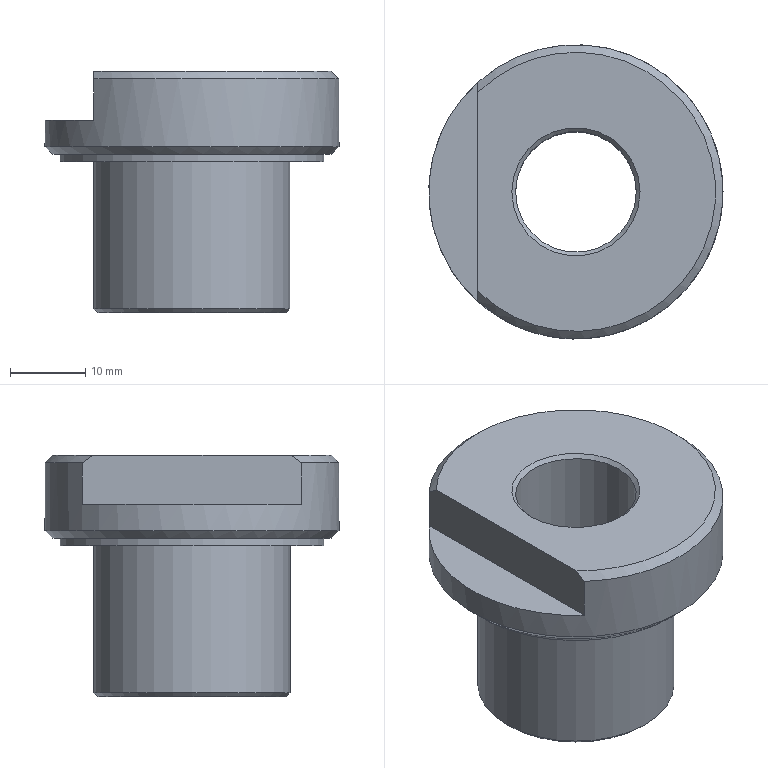Component | NX | DRILL_BUSHING | 1 solid | 17 faces | box 39 x 39 x 32 mm | volume 17133 mm3 | plane 7 | cylinder 5 | cone 5 | commonest cylinder face diameters 35 x1 39 x1 30 x1 26 x1 16 x1
STEP:
#1=CARTESIAN_POINT('',(0.,0.,0.));
#2=DIRECTION('',(0.,0.,1.));
#3=DIRECTION('',(1.,0.,0.));
#4=AXIS2_PLACEMENT_3D('',#1,#2,#3);
#5=CARTESIAN_POINT('',(30.5,0.,39.));
#6=VERTEX_POINT('',#5);
#7=CARTESIAN_POINT('',(13.,0.,39.));
#8=DIRECTION('',(0.,0.,1.));
#9=DIRECTION('',(1.,0.,0.));
#10=AXIS2_PLACEMENT_3D('',#7,#8,#9);
#11=CIRCLE('',#10,17.5);
#12=CARTESIAN_POINT('',(13.,0.,39.));
#13=DIRECTION('',(0.,0.,-1.));
#14=DIRECTION('',(-1.,0.,0.));
#15=AXIS2_PLACEMENT_3D('',#12,#13,#14);
#16=CYLINDRICAL_SURFACE('',#15,17.5);
#17=CARTESIAN_POINT('',(9.425,0.));
#18=DIRECTION('',(-1.,0.));
#19=VECTOR('',#18,1.);
#20=LINE('',#17,#19);
#21=(GEOMETRIC_REPRESENTATION_CONTEXT(2)PARAMETRIC_REPRESENTATION_CONTEXT()REPRESENTATION_CONTEXT('',''));
#22=DEFINITIONAL_REPRESENTATION('',(#20),#21);
#23=PCURVE('',#16,#22);
#24=CARTESIAN_POINT('',(13.,0.,39.));
#25=DIRECTION('',(0.,0.,1.));
#26=DIRECTION('',(1.,0.,0.));
#27=AXIS2_PLACEMENT_3D('',#24,#25,#26);
#28=PLANE('',#27);
#29=CARTESIAN_POINT('',(0.,0.));
#30=DIRECTION('',(1.,0.));
#31=AXIS2_PLACEMENT_2D('',#29,#30);
#32=CIRCLE('',#31,17.5);
#33=(GEOMETRIC_REPRESENTATION_CONTEXT(2)PARAMETRIC_REPRESENTATION_CONTEXT()REPRESENTATION_CONTEXT('',''));
#34=DEFINITIONAL_REPRESENTATION('',(#32),#33);
#35=PCURVE('',#28,#34);
#36=SURFACE_CURVE('',#11,(#23,#35),.PCURVE_S1.);
#37=EDGE_CURVE('',#6,#6,#36,.T.);
#38=ORIENTED_EDGE('',*,*,#37,.F.);
#39=CARTESIAN_POINT('',(30.5,0.,38.));
#40=VERTEX_POINT('',#39);
#41=CARTESIAN_POINT('',(30.5,0.,39.));
#42=CARTESIAN_POINT('',(30.5,0.,38.));
#43=B_SPLINE_CURVE_WITH_KNOTS('',1,(#41,#42),.UNSPECIFIED.,.F.,.F.,(2,2),(0.,1.),.PIECEWISE_BEZIER_KNOTS.);
#44=CARTESIAN_POINT('',(9.425,0.));
#45=DIRECTION('',(0.,1.));
#46=VECTOR('',#45,1.);
#47=LINE('',#44,#46);
#48=(GEOMETRIC_REPRESENTATION_CONTEXT(2)PARAMETRIC_REPRESENTATION_CONTEXT()REPRESENTATION_CONTEXT('',''));
#49=DEFINITIONAL_REPRESENTATION('',(#47),#48);
#50=PCURVE('',#16,#49);
#51=CARTESIAN_POINT('',(3.142,0.));
#52=DIRECTION('',(0.,1.));
#53=VECTOR('',#52,1.);
#54=LINE('',#51,#53);
#55=(GEOMETRIC_REPRESENTATION_CONTEXT(2)PARAMETRIC_REPRESENTATION_CONTEXT()REPRESENTATION_CONTEXT('',''));
#56=DEFINITIONAL_REPRESENTATION('',(#54),#55);
#57=PCURVE('',#16,#56);
#58=SEAM_CURVE('',#43,(#50,#57),.PCURVE_S1.);
#59=EDGE_CURVE('',#6,#40,#58,.T.);
#60=ORIENTED_EDGE('',*,*,#59,.T.);
#61=CARTESIAN_POINT('',(13.,0.,38.));
#62=DIRECTION('',(0.,0.,1.));
#63=DIRECTION('',(1.,0.,0.));
#64=AXIS2_PLACEMENT_3D('',#61,#62,#63);
#65=CIRCLE('',#64,17.5);
#66=CARTESIAN_POINT('',(9.425,1.));
#67=DIRECTION('',(-1.,0.));
#68=VECTOR('',#67,1.);
#69=LINE('',#66,#68);
#70=(GEOMETRIC_REPRESENTATION_CONTEXT(2)PARAMETRIC_REPRESENTATION_CONTEXT()REPRESENTATION_CONTEXT('',''));
#71=DEFINITIONAL_REPRESENTATION('',(#69),#70);
#72=PCURVE('',#16,#71);
#73=CARTESIAN_POINT('',(13.,0.,38.));
#74=DIRECTION('',(0.,0.,1.));
#75=DIRECTION('',(1.,0.,0.));
#76=AXIS2_PLACEMENT_3D('',#73,#74,#75);
#77=PLANE('',#76);
#78=CARTESIAN_POINT('',(0.,0.));
#79=DIRECTION('',(1.,0.));
#80=AXIS2_PLACEMENT_2D('',#78,#79);
#81=CIRCLE('',#80,17.5);
#82=(GEOMETRIC_REPRESENTATION_CONTEXT(2)PARAMETRIC_REPRESENTATION_CONTEXT()REPRESENTATION_CONTEXT('',''));
#83=DEFINITIONAL_REPRESENTATION('',(#81),#82);
#84=PCURVE('',#77,#83);
#85=SURFACE_CURVE('',#65,(#72,#84),.PCURVE_S1.);
#86=EDGE_CURVE('',#40,#40,#85,.T.);
#87=ORIENTED_EDGE('',*,*,#86,.T.);
#88=ORIENTED_EDGE('',*,*,#59,.F.);
#89=EDGE_LOOP('',(#38,#60,#87,#88));
#90=FACE_BOUND('',#89,.T.);
#91=ADVANCED_FACE('',(#90),#16,.T.);
#92=CARTESIAN_POINT('',(28.,0.,38.));
#93=VERTEX_POINT('',#92);
#94=CARTESIAN_POINT('',(13.,0.,38.));
#95=DIRECTION('',(0.,0.,-1.));
#96=DIRECTION('',(1.,0.,0.));
#97=AXIS2_PLACEMENT_3D('',#94,#95,#96);
#98=CIRCLE('',#97,15.);
#99=CARTESIAN_POINT('',(15.,0.));
#100=CARTESIAN_POINT('',(15.,-25.981));
#101=CARTESIAN_POINT('',(-7.5,-12.99));
#102=CARTESIAN_POINT('',(-30.,-0.));
#103=CARTESIAN_POINT('',(-7.5,12.99));
#104=CARTESIAN_POINT('',(15.,25.981));
#105=CARTESIAN_POINT('',(15.,0.));
#106=(BOUNDED_CURVE()B_SPLINE_CURVE(2,(#99,#100,#101,#102,#103,#104,#105),.UNSPECIFIED.,.T.,.F.)B_SPLINE_CURVE_WITH_KNOTS((1,2,2,2,2,1),(-2.094,0.,2.094,4.189,6.283,8.378),.UNSPECIFIED.)CURVE()GEOMETRIC_REPRESENTATION_ITEM()RATIONAL_B_SPLINE_CURVE((1.,0.5,1.,0.5,1.,0.5,1.))REPRESENTATION_ITEM(''));
#107=(GEOMETRIC_REPRESENTATION_CONTEXT(2)PARAMETRIC_REPRESENTATION_CONTEXT()REPRESENTATION_CONTEXT('',''));
#108=DEFINITIONAL_REPRESENTATION('',(#106),#107);
#109=PCURVE('',#77,#108);
#110=CARTESIAN_POINT('',(13.,0.,38.));
#111=DIRECTION('',(0.,0.,1.));
#112=DIRECTION('',(1.,0.,0.));
#113=AXIS2_PLACEMENT_3D('',#110,#111,#112);
#114=CYLINDRICAL_SURFACE('',#113,15.);
#115=CARTESIAN_POINT('',(6.283,0.));
#116=DIRECTION('',(-1.,0.));
#117=VECTOR('',#116,1.);
#118=LINE('',#115,#117);
#119=(GEOMETRIC_REPRESENTATION_CONTEXT(2)PARAMETRIC_REPRESENTATION_CONTEXT()REPRESENTATION_CONTEXT('',''));
#120=DEFINITIONAL_REPRESENTATION('',(#118),#119);
#121=PCURVE('',#114,#120);
#122=SURFACE_CURVE('',#98,(#109,#121),.PCURVE_S1.);
#123=EDGE_CURVE('',#93,#93,#122,.T.);
#124=ORIENTED_EDGE('',*,*,#123,.F.);
#125=EDGE_LOOP('',(#124));
#126=FACE_BOUND('',#125,.T.);
#127=ORIENTED_EDGE('',*,*,#86,.F.);
#128=EDGE_LOOP('',(#127));
#129=FACE_BOUND('',#128,.T.);
#130=ADVANCED_FACE('',(#126,#129),#77,.F.);
#131=CARTESIAN_POINT('',(32.5,0.,40.));
#132=VERTEX_POINT('',#131);
#133=CARTESIAN_POINT('',(-0.,14.534,40.));
#134=VERTEX_POINT('',#133);
#135=CARTESIAN_POINT('',(13.,0.,40.));
#136=DIRECTION('',(0.,0.,1.));
#137=DIRECTION('',(1.,0.,0.));
#138=AXIS2_PLACEMENT_3D('',#135,#136,#137);
#139=CIRCLE('',#138,19.5);
#140=CARTESIAN_POINT('',(13.,0.,50.));
#141=DIRECTION('',(0.,0.,-1.));
#142=DIRECTION('',(-1.,0.,0.));
#143=AXIS2_PLACEMENT_3D('',#140,#141,#142);
#144=CYLINDRICAL_SURFACE('',#143,19.5);
#145=CARTESIAN_POINT('',(3.142,10.));
#146=DIRECTION('',(-1.,0.));
#147=VECTOR('',#146,1.);
#148=LINE('',#145,#147);
#149=(GEOMETRIC_REPRESENTATION_CONTEXT(2)PARAMETRIC_REPRESENTATION_CONTEXT()REPRESENTATION_CONTEXT('',''));
#150=DEFINITIONAL_REPRESENTATION('',(#148),#149);
#151=PCURVE('',#144,#150);
#152=CARTESIAN_POINT('',(13.,0.,40.));
#153=DIRECTION('',(0.,0.,1.));
#154=DIRECTION('',(1.,0.,0.));
#155=AXIS2_PLACEMENT_3D('',#152,#153,#154);
#156=CONICAL_SURFACE('',#155,19.5,0.7854);
#157=CARTESIAN_POINT('',(0.,0.));
#158=DIRECTION('',(1.,0.));
#159=VECTOR('',#158,1.);
#160=LINE('',#157,#159);
#161=(GEOMETRIC_REPRESENTATION_CONTEXT(2)PARAMETRIC_REPRESENTATION_CONTEXT()REPRESENTATION_CONTEXT('',''));
#162=DEFINITIONAL_REPRESENTATION('',(#160),#161);
#163=PCURVE('',#156,#162);
#164=SURFACE_CURVE('',#139,(#151,#163),.PCURVE_S1.);
#165=EDGE_CURVE('',#132,#134,#164,.T.);
#166=ORIENTED_EDGE('',*,*,#165,.T.);
#167=CARTESIAN_POINT('',(0.,14.534,43.5));
#168=VERTEX_POINT('',#167);
#169=CARTESIAN_POINT('',(-0.,14.534,43.5));
#170=CARTESIAN_POINT('',(-0.,14.534,40.));
#171=B_SPLINE_CURVE_WITH_KNOTS('',1,(#169,#170),.UNSPECIFIED.,.F.,.F.,(2,2),(6.5,10.),.PIECEWISE_BEZIER_KNOTS.);
#172=CARTESIAN_POINT('',(0.8411,0.));
#173=DIRECTION('',(0.,1.));
#174=VECTOR('',#173,1.);
#175=LINE('',#172,#174);
#176=(GEOMETRIC_REPRESENTATION_CONTEXT(2)PARAMETRIC_REPRESENTATION_CONTEXT()REPRESENTATION_CONTEXT('',''));
#177=DEFINITIONAL_REPRESENTATION('',(#175),#176);
#178=PCURVE('',#144,#177);
#179=CARTESIAN_POINT('',(7.124,0.));
#180=DIRECTION('',(0.,1.));
#181=VECTOR('',#180,1.);
#182=LINE('',#179,#181);
#183=(GEOMETRIC_REPRESENTATION_CONTEXT(2)PARAMETRIC_REPRESENTATION_CONTEXT()REPRESENTATION_CONTEXT('',''));
#184=DEFINITIONAL_REPRESENTATION('',(#182),#183);
#185=PCURVE('',#144,#184);
#186=SEAM_CURVE('',#171,(#178,#185),.PCURVE_S1.);
#187=EDGE_CURVE('',#168,#134,#186,.T.);
#188=ORIENTED_EDGE('',*,*,#187,.F.);
#189=CARTESIAN_POINT('',(0.,14.534,49.));
#190=VERTEX_POINT('',#189);
#191=CARTESIAN_POINT('',(0.,14.534,50.));
#192=DIRECTION('',(0.,0.,1.));
#193=VECTOR('',#192,1.);
#194=LINE('',#191,#193);
#195=CARTESIAN_POINT('',(0.8411,0.));
#196=DIRECTION('',(0.,-1.));
#197=VECTOR('',#196,1.);
#198=LINE('',#195,#197);
#199=(GEOMETRIC_REPRESENTATION_CONTEXT(2)PARAMETRIC_REPRESENTATION_CONTEXT()REPRESENTATION_CONTEXT('',''));
#200=DEFINITIONAL_REPRESENTATION('',(#198),#199);
#201=PCURVE('',#144,#200);
#202=CARTESIAN_POINT('',(0.,-23.,43.5));
#203=DIRECTION('',(1.,0.,0.));
#204=DIRECTION('',(-0.,1.,0.));
#205=AXIS2_PLACEMENT_3D('',#202,#203,#204);
#206=PLANE('',#205);
#207=CARTESIAN_POINT('',(37.534,6.5));
#208=DIRECTION('',(0.,1.));
#209=VECTOR('',#208,1.);
#210=LINE('',#207,#209);
#211=(GEOMETRIC_REPRESENTATION_CONTEXT(2)PARAMETRIC_REPRESENTATION_CONTEXT()REPRESENTATION_CONTEXT('',''));
#212=DEFINITIONAL_REPRESENTATION('',(#210),#211);
#213=PCURVE('',#206,#212);
#214=SURFACE_CURVE('',#194,(#201,#213),.PCURVE_S1.);
#215=EDGE_CURVE('',#168,#190,#214,.T.);
#216=ORIENTED_EDGE('',*,*,#215,.T.);
#217=CARTESIAN_POINT('',(0.,-14.534,49.));
#218=VERTEX_POINT('',#217);
#219=CARTESIAN_POINT('',(13.,0.,49.));
#220=DIRECTION('',(0.,0.,-1.));
#221=DIRECTION('',(1.,0.,0.));
#222=AXIS2_PLACEMENT_3D('',#219,#220,#221);
#223=CIRCLE('',#222,19.5);
#224=CARTESIAN_POINT('',(-3.142,1.));
#225=DIRECTION('',(1.,0.));
#226=VECTOR('',#225,1.);
#227=LINE('',#224,#226);
#228=(GEOMETRIC_REPRESENTATION_CONTEXT(2)PARAMETRIC_REPRESENTATION_CONTEXT()REPRESENTATION_CONTEXT('',''));
#229=DEFINITIONAL_REPRESENTATION('',(#227),#228);
#230=PCURVE('',#144,#229);
#231=CARTESIAN_POINT('',(13.,0.,50.));
#232=DIRECTION('',(0.,0.,-1.));
#233=DIRECTION('',(-1.,0.,0.));
#234=AXIS2_PLACEMENT_3D('',#231,#232,#233);
#235=CONICAL_SURFACE('',#234,18.5,0.7854);
#236=CARTESIAN_POINT('',(-3.142,1.));
#237=DIRECTION('',(1.,0.));
#238=VECTOR('',#237,1.);
#239=LINE('',#236,#238);
#240=(GEOMETRIC_REPRESENTATION_CONTEXT(2)PARAMETRIC_REPRESENTATION_CONTEXT()REPRESENTATION_CONTEXT('',''));
#241=DEFINITIONAL_REPRESENTATION('',(#239),#240);
#242=PCURVE('',#235,#241);
#243=SURFACE_CURVE('',#223,(#230,#242),.PCURVE_S1.);
#244=EDGE_CURVE('',#190,#218,#243,.T.);
#245=ORIENTED_EDGE('',*,*,#244,.T.);
#246=CARTESIAN_POINT('',(0.,-14.534,43.5));
#247=VERTEX_POINT('',#246);
#248=CARTESIAN_POINT('',(0.,-14.534,50.));
#249=DIRECTION('',(0.,0.,-1.));
#250=VECTOR('',#249,1.);
#251=LINE('',#248,#250);
#252=CARTESIAN_POINT('',(5.442,0.));
#253=DIRECTION('',(0.,1.));
#254=VECTOR('',#253,1.);
#255=LINE('',#252,#254);
#256=(GEOMETRIC_REPRESENTATION_CONTEXT(2)PARAMETRIC_REPRESENTATION_CONTEXT()REPRESENTATION_CONTEXT('',''));
#257=DEFINITIONAL_REPRESENTATION('',(#255),#256);
#258=PCURVE('',#144,#257);
#259=CARTESIAN_POINT('',(8.466,6.5));
#260=DIRECTION('',(0.,-1.));
#261=VECTOR('',#260,1.);
#262=LINE('',#259,#261);
#263=(GEOMETRIC_REPRESENTATION_CONTEXT(2)PARAMETRIC_REPRESENTATION_CONTEXT()REPRESENTATION_CONTEXT('',''));
#264=DEFINITIONAL_REPRESENTATION('',(#262),#263);
#265=PCURVE('',#206,#264);
#266=SURFACE_CURVE('',#251,(#258,#265),.PCURVE_S1.);
#267=EDGE_CURVE('',#218,#247,#266,.T.);
#268=ORIENTED_EDGE('',*,*,#267,.T.);
#269=CARTESIAN_POINT('',(13.,0.,43.5));
#270=DIRECTION('',(0.,0.,1.));
#271=DIRECTION('',(1.,0.,0.));
#272=AXIS2_PLACEMENT_3D('',#269,#270,#271);
#273=CIRCLE('',#272,19.5);
#274=CARTESIAN_POINT('',(9.425,6.5));
#275=DIRECTION('',(-1.,0.));
#276=VECTOR('',#275,1.);
#277=LINE('',#274,#276);
#278=(GEOMETRIC_REPRESENTATION_CONTEXT(2)PARAMETRIC_REPRESENTATION_CONTEXT()REPRESENTATION_CONTEXT('',''));
#279=DEFINITIONAL_REPRESENTATION('',(#277),#278);
#280=PCURVE('',#144,#279);
#281=CARTESIAN_POINT('',(13.,0.,43.5));
#282=DIRECTION('',(0.,0.,1.));
#283=DIRECTION('',(1.,0.,0.));
#284=AXIS2_PLACEMENT_3D('',#281,#282,#283);
#285=PLANE('',#284);
#286=CARTESIAN_POINT('',(0.,0.));
#287=DIRECTION('',(1.,0.));
#288=AXIS2_PLACEMENT_2D('',#286,#287);
#289=CIRCLE('',#288,19.5);
#290=(GEOMETRIC_REPRESENTATION_CONTEXT(2)PARAMETRIC_REPRESENTATION_CONTEXT()REPRESENTATION_CONTEXT('',''));
#291=DEFINITIONAL_REPRESENTATION('',(#289),#290);
#292=PCURVE('',#285,#291);
#293=SURFACE_CURVE('',#273,(#280,#292),.PCURVE_S1.);
#294=EDGE_CURVE('',#168,#247,#293,.T.);
#295=ORIENTED_EDGE('',*,*,#294,.F.);
#296=ORIENTED_EDGE('',*,*,#187,.T.);
#297=CARTESIAN_POINT('',(13.,0.,40.));
#298=DIRECTION('',(0.,0.,1.));
#299=DIRECTION('',(1.,0.,0.));
#300=AXIS2_PLACEMENT_3D('',#297,#298,#299);
#301=CIRCLE('',#300,19.5);
#302=CARTESIAN_POINT('',(9.425,10.));
#303=DIRECTION('',(-1.,0.));
#304=VECTOR('',#303,1.);
#305=LINE('',#302,#304);
#306=(GEOMETRIC_REPRESENTATION_CONTEXT(2)PARAMETRIC_REPRESENTATION_CONTEXT()REPRESENTATION_CONTEXT('',''));
#307=DEFINITIONAL_REPRESENTATION('',(#305),#306);
#308=PCURVE('',#144,#307);
#309=CARTESIAN_POINT('',(0.,0.));
#310=DIRECTION('',(1.,0.));
#311=VECTOR('',#310,1.);
#312=LINE('',#309,#311);
#313=(GEOMETRIC_REPRESENTATION_CONTEXT(2)PARAMETRIC_REPRESENTATION_CONTEXT()REPRESENTATION_CONTEXT('',''));
#314=DEFINITIONAL_REPRESENTATION('',(#312),#313);
#315=PCURVE('',#156,#314);
#316=SURFACE_CURVE('',#301,(#308,#315),.PCURVE_S1.);
#317=EDGE_CURVE('',#134,#132,#316,.T.);
#318=ORIENTED_EDGE('',*,*,#317,.T.);
#319=EDGE_LOOP('',(#166,#188,#216,#245,#268,#295,#296,#318));
#320=FACE_BOUND('',#319,.T.);
#321=ADVANCED_FACE('',(#320),#144,.T.);
#322=CARTESIAN_POINT('',(21.5,0.,50.));
#323=VERTEX_POINT('',#322);
#324=CARTESIAN_POINT('',(13.,0.,50.));
#325=DIRECTION('',(0.,0.,-1.));
#326=DIRECTION('',(1.,0.,0.));
#327=AXIS2_PLACEMENT_3D('',#324,#325,#326);
#328=CIRCLE('',#327,8.5);
#329=CARTESIAN_POINT('',(13.,0.,50.));
#330=DIRECTION('',(0.,0.,1.));
#331=DIRECTION('',(1.,0.,0.));
#332=AXIS2_PLACEMENT_3D('',#329,#330,#331);
#333=PLANE('',#332);
#334=CARTESIAN_POINT('',(8.5,0.));
#335=CARTESIAN_POINT('',(8.5,-14.722));
#336=CARTESIAN_POINT('',(-4.25,-7.361));
#337=CARTESIAN_POINT('',(-17.,-0.));
#338=CARTESIAN_POINT('',(-4.25,7.361));
#339=CARTESIAN_POINT('',(8.5,14.722));
#340=CARTESIAN_POINT('',(8.5,0.));
#341=(BOUNDED_CURVE()B_SPLINE_CURVE(2,(#334,#335,#336,#337,#338,#339,#340),.UNSPECIFIED.,.T.,.F.)B_SPLINE_CURVE_WITH_KNOTS((1,2,2,2,2,1),(-2.094,0.,2.094,4.189,6.283,8.378),.UNSPECIFIED.)CURVE()GEOMETRIC_REPRESENTATION_ITEM()RATIONAL_B_SPLINE_CURVE((1.,0.5,1.,0.5,1.,0.5,1.))REPRESENTATION_ITEM(''));
#342=(GEOMETRIC_REPRESENTATION_CONTEXT(2)PARAMETRIC_REPRESENTATION_CONTEXT()REPRESENTATION_CONTEXT('',''));
#343=DEFINITIONAL_REPRESENTATION('',(#341),#342);
#344=PCURVE('',#333,#343);
#345=CARTESIAN_POINT('',(13.,0.,50.));
#346=DIRECTION('',(0.,0.,1.));
#347=DIRECTION('',(1.,0.,0.));
#348=AXIS2_PLACEMENT_3D('',#345,#346,#347);
#349=CONICAL_SURFACE('',#348,8.5,0.7854);
#350=CARTESIAN_POINT('',(6.283,0.));
#351=DIRECTION('',(-1.,0.));
#352=VECTOR('',#351,1.);
#353=LINE('',#350,#352);
#354=(GEOMETRIC_REPRESENTATION_CONTEXT(2)PARAMETRIC_REPRESENTATION_CONTEXT()REPRESENTATION_CONTEXT('',''));
#355=DEFINITIONAL_REPRESENTATION('',(#353),#354);
#356=PCURVE('',#349,#355);
#357=SURFACE_CURVE('',#328,(#344,#356),.PCURVE_S1.);
#358=EDGE_CURVE('',#323,#323,#357,.T.);
#359=ORIENTED_EDGE('',*,*,#358,.T.);
#360=EDGE_LOOP('',(#359));
#361=FACE_BOUND('',#360,.T.);
#362=CARTESIAN_POINT('',(0.,-13.162,50.));
#363=VERTEX_POINT('',#362);
#364=CARTESIAN_POINT('',(0.,13.162,50.));
#365=VERTEX_POINT('',#364);
#366=CARTESIAN_POINT('',(0.,-23.,50.));
#367=DIRECTION('',(-0.,1.,0.));
#368=VECTOR('',#367,1.);
#369=LINE('',#366,#368);
#370=CARTESIAN_POINT('',(-13.,-23.));
#371=DIRECTION('',(-0.,1.));
#372=VECTOR('',#371,1.);
#373=LINE('',#370,#372);
#374=(GEOMETRIC_REPRESENTATION_CONTEXT(2)PARAMETRIC_REPRESENTATION_CONTEXT()REPRESENTATION_CONTEXT('',''));
#375=DEFINITIONAL_REPRESENTATION('',(#373),#374);
#376=PCURVE('',#333,#375);
#377=CARTESIAN_POINT('',(0.,6.5));
#378=DIRECTION('',(1.,0.));
#379=VECTOR('',#378,1.);
#380=LINE('',#377,#379);
#381=(GEOMETRIC_REPRESENTATION_CONTEXT(2)PARAMETRIC_REPRESENTATION_CONTEXT()REPRESENTATION_CONTEXT('',''));
#382=DEFINITIONAL_REPRESENTATION('',(#380),#381);
#383=PCURVE('',#206,#382);
#384=SURFACE_CURVE('',#369,(#376,#383),.PCURVE_S1.);
#385=EDGE_CURVE('',#363,#365,#384,.T.);
#386=ORIENTED_EDGE('',*,*,#385,.F.);
#387=CARTESIAN_POINT('',(13.,0.,50.));
#388=DIRECTION('',(0.,0.,1.));
#389=DIRECTION('',(1.,0.,0.));
#390=AXIS2_PLACEMENT_3D('',#387,#388,#389);
#391=CIRCLE('',#390,18.5);
#392=CARTESIAN_POINT('',(0.,0.));
#393=DIRECTION('',(1.,0.));
#394=AXIS2_PLACEMENT_2D('',#392,#393);
#395=CIRCLE('',#394,18.5);
#396=(GEOMETRIC_REPRESENTATION_CONTEXT(2)PARAMETRIC_REPRESENTATION_CONTEXT()REPRESENTATION_CONTEXT('',''));
#397=DEFINITIONAL_REPRESENTATION('',(#395),#396);
#398=PCURVE('',#333,#397);
#399=CARTESIAN_POINT('',(9.425,0.));
#400=DIRECTION('',(-1.,0.));
#401=VECTOR('',#400,1.);
#402=LINE('',#399,#401);
#403=(GEOMETRIC_REPRESENTATION_CONTEXT(2)PARAMETRIC_REPRESENTATION_CONTEXT()REPRESENTATION_CONTEXT('',''));
#404=DEFINITIONAL_REPRESENTATION('',(#402),#403);
#405=PCURVE('',#235,#404);
#406=SURFACE_CURVE('',#391,(#398,#405),.PCURVE_S1.);
#407=EDGE_CURVE('',#363,#365,#406,.T.);
#408=ORIENTED_EDGE('',*,*,#407,.T.);
#409=EDGE_LOOP('',(#386,#408));
#410=FACE_BOUND('',#409,.T.);
#411=ADVANCED_FACE('',(#361,#410),#333,.T.);
#412=CARTESIAN_POINT('',(31.5,0.,39.));
#413=VERTEX_POINT('',#412);
#414=CARTESIAN_POINT('',(13.,0.,39.));
#415=DIRECTION('',(0.,0.,-1.));
#416=DIRECTION('',(1.,0.,0.));
#417=AXIS2_PLACEMENT_3D('',#414,#415,#416);
#418=CIRCLE('',#417,18.5);
#419=CARTESIAN_POINT('',(18.5,0.));
#420=CARTESIAN_POINT('',(18.5,-32.043));
#421=CARTESIAN_POINT('',(-9.25,-16.021));
#422=CARTESIAN_POINT('',(-37.,-0.));
#423=CARTESIAN_POINT('',(-9.25,16.021));
#424=CARTESIAN_POINT('',(18.5,32.043));
#425=CARTESIAN_POINT('',(18.5,0.));
#426=(BOUNDED_CURVE()B_SPLINE_CURVE(2,(#419,#420,#421,#422,#423,#424,#425),.UNSPECIFIED.,.T.,.F.)B_SPLINE_CURVE_WITH_KNOTS((1,2,2,2,2,1),(-2.094,0.,2.094,4.189,6.283,8.378),.UNSPECIFIED.)CURVE()GEOMETRIC_REPRESENTATION_ITEM()RATIONAL_B_SPLINE_CURVE((1.,0.5,1.,0.5,1.,0.5,1.))REPRESENTATION_ITEM(''));
#427=(GEOMETRIC_REPRESENTATION_CONTEXT(2)PARAMETRIC_REPRESENTATION_CONTEXT()REPRESENTATION_CONTEXT('',''));
#428=DEFINITIONAL_REPRESENTATION('',(#426),#427);
#429=PCURVE('',#28,#428);
#430=CARTESIAN_POINT('',(6.283,-1.));
#431=DIRECTION('',(-1.,0.));
#432=VECTOR('',#431,1.);
#433=LINE('',#430,#432);
#434=(GEOMETRIC_REPRESENTATION_CONTEXT(2)PARAMETRIC_REPRESENTATION_CONTEXT()REPRESENTATION_CONTEXT('',''));
#435=DEFINITIONAL_REPRESENTATION('',(#433),#434);
#436=PCURVE('',#156,#435);
#437=SURFACE_CURVE('',#418,(#429,#436),.PCURVE_S1.);
#438=EDGE_CURVE('',#413,#413,#437,.T.);
#439=ORIENTED_EDGE('',*,*,#438,.T.);
#440=EDGE_LOOP('',(#439));
#441=FACE_BOUND('',#440,.T.);
#442=ORIENTED_EDGE('',*,*,#37,.T.);
#443=EDGE_LOOP('',(#442));
#444=FACE_BOUND('',#443,.T.);
#445=ADVANCED_FACE('',(#441,#444),#28,.F.);
#446=CARTESIAN_POINT('',(28.,0.,39.));
#447=VERTEX_POINT('',#446);
#448=CARTESIAN_POINT('',(13.,0.,39.));
#449=DIRECTION('',(0.,0.,1.));
#450=DIRECTION('',(1.,0.,0.));
#451=AXIS2_PLACEMENT_3D('',#448,#449,#450);
#452=CIRCLE('',#451,15.);
#453=CARTESIAN_POINT('',(13.,0.,39.));
#454=DIRECTION('',(0.,0.,1.));
#455=DIRECTION('',(1.,0.,0.));
#456=AXIS2_PLACEMENT_3D('',#453,#454,#455);
#457=PLANE('',#456);
#458=CARTESIAN_POINT('',(0.,0.));
#459=DIRECTION('',(1.,0.));
#460=AXIS2_PLACEMENT_2D('',#458,#459);
#461=CIRCLE('',#460,15.);
#462=(GEOMETRIC_REPRESENTATION_CONTEXT(2)PARAMETRIC_REPRESENTATION_CONTEXT()REPRESENTATION_CONTEXT('',''));
#463=DEFINITIONAL_REPRESENTATION('',(#461),#462);
#464=PCURVE('',#457,#463);
#465=CARTESIAN_POINT('',(0.,1.));
#466=DIRECTION('',(1.,0.));
#467=VECTOR('',#466,1.);
#468=LINE('',#465,#467);
#469=(GEOMETRIC_REPRESENTATION_CONTEXT(2)PARAMETRIC_REPRESENTATION_CONTEXT()REPRESENTATION_CONTEXT('',''));
#470=DEFINITIONAL_REPRESENTATION('',(#468),#469);
#471=PCURVE('',#114,#470);
#472=SURFACE_CURVE('',#452,(#464,#471),.PCURVE_S1.);
#473=EDGE_CURVE('',#447,#447,#472,.T.);
#474=ORIENTED_EDGE('',*,*,#473,.F.);
#475=EDGE_LOOP('',(#474));
#476=FACE_BOUND('',#475,.T.);
#477=CARTESIAN_POINT('',(26.,0.,39.));
#478=VERTEX_POINT('',#477);
#479=CARTESIAN_POINT('',(13.,0.,39.));
#480=DIRECTION('',(0.,0.,-1.));
#481=DIRECTION('',(1.,0.,0.));
#482=AXIS2_PLACEMENT_3D('',#479,#480,#481);
#483=CIRCLE('',#482,13.);
#484=CARTESIAN_POINT('',(13.,0.));
#485=CARTESIAN_POINT('',(13.,-22.517));
#486=CARTESIAN_POINT('',(-6.5,-11.258));
#487=CARTESIAN_POINT('',(-26.,-0.));
#488=CARTESIAN_POINT('',(-6.5,11.258));
#489=CARTESIAN_POINT('',(13.,22.517));
#490=CARTESIAN_POINT('',(13.,0.));
#491=(BOUNDED_CURVE()B_SPLINE_CURVE(2,(#484,#485,#486,#487,#488,#489,#490),.UNSPECIFIED.,.T.,.F.)B_SPLINE_CURVE_WITH_KNOTS((1,2,2,2,2,1),(-2.094,0.,2.094,4.189,6.283,8.378),.UNSPECIFIED.)CURVE()GEOMETRIC_REPRESENTATION_ITEM()RATIONAL_B_SPLINE_CURVE((1.,0.5,1.,0.5,1.,0.5,1.))REPRESENTATION_ITEM(''));
#492=(GEOMETRIC_REPRESENTATION_CONTEXT(2)PARAMETRIC_REPRESENTATION_CONTEXT()REPRESENTATION_CONTEXT('',''));
#493=DEFINITIONAL_REPRESENTATION('',(#491),#492);
#494=PCURVE('',#457,#493);
#495=CARTESIAN_POINT('',(13.,0.,38.));
#496=DIRECTION('',(0.,0.,-1.));
#497=DIRECTION('',(-1.,0.,0.));
#498=AXIS2_PLACEMENT_3D('',#495,#496,#497);
#499=CYLINDRICAL_SURFACE('',#498,13.);
#500=CARTESIAN_POINT('',(3.142,-1.));
#501=DIRECTION('',(1.,0.));
#502=VECTOR('',#501,1.);
#503=LINE('',#500,#502);
#504=(GEOMETRIC_REPRESENTATION_CONTEXT(2)PARAMETRIC_REPRESENTATION_CONTEXT()REPRESENTATION_CONTEXT('',''));
#505=DEFINITIONAL_REPRESENTATION('',(#503),#504);
#506=PCURVE('',#499,#505);
#507=SURFACE_CURVE('',#483,(#494,#506),.PCURVE_S1.);
#508=EDGE_CURVE('',#478,#478,#507,.T.);
#509=ORIENTED_EDGE('',*,*,#508,.F.);
#510=EDGE_LOOP('',(#509));
#511=FACE_BOUND('',#510,.T.);
#512=ADVANCED_FACE('',(#476,#511),#457,.F.);
#513=ORIENTED_EDGE('',*,*,#123,.F.);
#514=CARTESIAN_POINT('',(28.,0.,38.));
#515=CARTESIAN_POINT('',(28.,0.,39.));
#516=B_SPLINE_CURVE_WITH_KNOTS('',1,(#514,#515),.UNSPECIFIED.,.F.,.F.,(2,2),(0.,1.),.PIECEWISE_BEZIER_KNOTS.);
#517=CARTESIAN_POINT('',(6.283,0.));
#518=DIRECTION('',(0.,1.));
#519=VECTOR('',#518,1.);
#520=LINE('',#517,#519);
#521=(GEOMETRIC_REPRESENTATION_CONTEXT(2)PARAMETRIC_REPRESENTATION_CONTEXT()REPRESENTATION_CONTEXT('',''));
#522=DEFINITIONAL_REPRESENTATION('',(#520),#521);
#523=PCURVE('',#114,#522);
#524=CARTESIAN_POINT('',(0.,0.));
#525=DIRECTION('',(0.,1.));
#526=VECTOR('',#525,1.);
#527=LINE('',#524,#526);
#528=(GEOMETRIC_REPRESENTATION_CONTEXT(2)PARAMETRIC_REPRESENTATION_CONTEXT()REPRESENTATION_CONTEXT('',''));
#529=DEFINITIONAL_REPRESENTATION('',(#527),#528);
#530=PCURVE('',#114,#529);
#531=SEAM_CURVE('',#516,(#523,#530),.PCURVE_S1.);
#532=EDGE_CURVE('',#93,#447,#531,.T.);
#533=ORIENTED_EDGE('',*,*,#532,.T.);
#534=ORIENTED_EDGE('',*,*,#473,.F.);
#535=ORIENTED_EDGE('',*,*,#532,.F.);
#536=EDGE_LOOP('',(#513,#533,#534,#535));
#537=FACE_BOUND('',#536,.F.);
#538=ADVANCED_FACE('',(#537),#114,.F.);
#539=CARTESIAN_POINT('',(21.5,0.,18.));
#540=VERTEX_POINT('',#539);
#541=CARTESIAN_POINT('',(13.,0.,18.));
#542=DIRECTION('',(0.,0.,1.));
#543=DIRECTION('',(1.,0.,0.));
#544=AXIS2_PLACEMENT_3D('',#541,#542,#543);
#545=CIRCLE('',#544,8.5);
#546=CARTESIAN_POINT('',(13.,0.,18.));
#547=DIRECTION('',(0.,0.,1.));
#548=DIRECTION('',(1.,0.,0.));
#549=AXIS2_PLACEMENT_3D('',#546,#547,#548);
#550=PLANE('',#549);
#551=CARTESIAN_POINT('',(0.,0.));
#552=DIRECTION('',(1.,0.));
#553=AXIS2_PLACEMENT_2D('',#551,#552);
#554=CIRCLE('',#553,8.5);
#555=(GEOMETRIC_REPRESENTATION_CONTEXT(2)PARAMETRIC_REPRESENTATION_CONTEXT()REPRESENTATION_CONTEXT('',''));
#556=DEFINITIONAL_REPRESENTATION('',(#554),#555);
#557=PCURVE('',#550,#556);
#558=CARTESIAN_POINT('',(13.,0.,18.));
#559=DIRECTION('',(0.,0.,-1.));
#560=DIRECTION('',(-1.,0.,0.));
#561=AXIS2_PLACEMENT_3D('',#558,#559,#560);
#562=CONICAL_SURFACE('',#561,8.5,0.7854);
#563=CARTESIAN_POINT('',(9.425,0.));
#564=DIRECTION('',(-1.,0.));
#565=VECTOR('',#564,1.);
#566=LINE('',#563,#565);
#567=(GEOMETRIC_REPRESENTATION_CONTEXT(2)PARAMETRIC_REPRESENTATION_CONTEXT()REPRESENTATION_CONTEXT('',''));
#568=DEFINITIONAL_REPRESENTATION('',(#566),#567);
#569=PCURVE('',#562,#568);
#570=SURFACE_CURVE('',#545,(#557,#569),.PCURVE_S1.);
#571=EDGE_CURVE('',#540,#540,#570,.T.);
#572=ORIENTED_EDGE('',*,*,#571,.T.);
#573=EDGE_LOOP('',(#572));
#574=FACE_BOUND('',#573,.T.);
#575=CARTESIAN_POINT('',(25.5,0.,18.));
#576=VERTEX_POINT('',#575);
#577=CARTESIAN_POINT('',(13.,0.,18.));
#578=DIRECTION('',(0.,0.,-1.));
#579=DIRECTION('',(1.,0.,0.));
#580=AXIS2_PLACEMENT_3D('',#577,#578,#579);
#581=CIRCLE('',#580,12.5);
#582=CARTESIAN_POINT('',(12.5,0.));
#583=CARTESIAN_POINT('',(12.5,-21.651));
#584=CARTESIAN_POINT('',(-6.25,-10.825));
#585=CARTESIAN_POINT('',(-25.,-0.));
#586=CARTESIAN_POINT('',(-6.25,10.825));
#587=CARTESIAN_POINT('',(12.5,21.651));
#588=CARTESIAN_POINT('',(12.5,0.));
#589=(BOUNDED_CURVE()B_SPLINE_CURVE(2,(#582,#583,#584,#585,#586,#587,#588),.UNSPECIFIED.,.T.,.F.)B_SPLINE_CURVE_WITH_KNOTS((1,2,2,2,2,1),(-2.094,0.,2.094,4.189,6.283,8.378),.UNSPECIFIED.)CURVE()GEOMETRIC_REPRESENTATION_ITEM()RATIONAL_B_SPLINE_CURVE((1.,0.5,1.,0.5,1.,0.5,1.))REPRESENTATION_ITEM(''));
#590=(GEOMETRIC_REPRESENTATION_CONTEXT(2)PARAMETRIC_REPRESENTATION_CONTEXT()REPRESENTATION_CONTEXT('',''));
#591=DEFINITIONAL_REPRESENTATION('',(#589),#590);
#592=PCURVE('',#550,#591);
#593=CARTESIAN_POINT('',(13.,0.,18.5));
#594=DIRECTION('',(0.,0.,1.));
#595=DIRECTION('',(1.,0.,0.));
#596=AXIS2_PLACEMENT_3D('',#593,#594,#595);
#597=CONICAL_SURFACE('',#596,13.,0.7854);
#598=CARTESIAN_POINT('',(6.283,-0.5));
#599=DIRECTION('',(-1.,0.));
#600=VECTOR('',#599,1.);
#601=LINE('',#598,#600);
#602=(GEOMETRIC_REPRESENTATION_CONTEXT(2)PARAMETRIC_REPRESENTATION_CONTEXT()REPRESENTATION_CONTEXT('',''));
#603=DEFINITIONAL_REPRESENTATION('',(#601),#602);
#604=PCURVE('',#597,#603);
#605=SURFACE_CURVE('',#581,(#592,#604),.PCURVE_S1.);
#606=EDGE_CURVE('',#576,#576,#605,.T.);
#607=ORIENTED_EDGE('',*,*,#606,.T.);
#608=EDGE_LOOP('',(#607));
#609=FACE_BOUND('',#608,.T.);
#610=ADVANCED_FACE('',(#574,#609),#550,.F.);
#611=CARTESIAN_POINT('',(26.,0.,18.5));
#612=VERTEX_POINT('',#611);
#613=CARTESIAN_POINT('',(13.,0.,18.5));
#614=DIRECTION('',(0.,0.,1.));
#615=DIRECTION('',(1.,0.,0.));
#616=AXIS2_PLACEMENT_3D('',#613,#614,#615);
#617=CIRCLE('',#616,13.);
#618=CARTESIAN_POINT('',(9.425,19.5));
#619=DIRECTION('',(-1.,0.));
#620=VECTOR('',#619,1.);
#621=LINE('',#618,#620);
#622=(GEOMETRIC_REPRESENTATION_CONTEXT(2)PARAMETRIC_REPRESENTATION_CONTEXT()REPRESENTATION_CONTEXT('',''));
#623=DEFINITIONAL_REPRESENTATION('',(#621),#622);
#624=PCURVE('',#499,#623);
#625=CARTESIAN_POINT('',(0.,0.));
#626=DIRECTION('',(1.,0.));
#627=VECTOR('',#626,1.);
#628=LINE('',#625,#627);
#629=(GEOMETRIC_REPRESENTATION_CONTEXT(2)PARAMETRIC_REPRESENTATION_CONTEXT()REPRESENTATION_CONTEXT('',''));
#630=DEFINITIONAL_REPRESENTATION('',(#628),#629);
#631=PCURVE('',#597,#630);
#632=SURFACE_CURVE('',#617,(#624,#631),.PCURVE_S1.);
#633=EDGE_CURVE('',#612,#612,#632,.T.);
#634=ORIENTED_EDGE('',*,*,#633,.T.);
#635=CARTESIAN_POINT('',(26.,0.,39.));
#636=CARTESIAN_POINT('',(26.,0.,18.5));
#637=B_SPLINE_CURVE_WITH_KNOTS('',1,(#635,#636),.UNSPECIFIED.,.F.,.F.,(2,2),(-1.,19.5),.PIECEWISE_BEZIER_KNOTS.);
#638=CARTESIAN_POINT('',(3.142,0.));
#639=DIRECTION('',(0.,1.));
#640=VECTOR('',#639,1.);
#641=LINE('',#638,#640);
#642=(GEOMETRIC_REPRESENTATION_CONTEXT(2)PARAMETRIC_REPRESENTATION_CONTEXT()REPRESENTATION_CONTEXT('',''));
#643=DEFINITIONAL_REPRESENTATION('',(#641),#642);
#644=PCURVE('',#499,#643);
#645=CARTESIAN_POINT('',(9.425,0.));
#646=DIRECTION('',(0.,1.));
#647=VECTOR('',#646,1.);
#648=LINE('',#645,#647);
#649=(GEOMETRIC_REPRESENTATION_CONTEXT(2)PARAMETRIC_REPRESENTATION_CONTEXT()REPRESENTATION_CONTEXT('',''));
#650=DEFINITIONAL_REPRESENTATION('',(#648),#649);
#651=PCURVE('',#499,#650);
#652=SEAM_CURVE('',#637,(#644,#651),.PCURVE_S1.);
#653=EDGE_CURVE('',#478,#612,#652,.T.);
#654=ORIENTED_EDGE('',*,*,#653,.F.);
#655=ORIENTED_EDGE('',*,*,#508,.T.);
#656=ORIENTED_EDGE('',*,*,#653,.T.);
#657=EDGE_LOOP('',(#634,#654,#655,#656));
#658=FACE_BOUND('',#657,.T.);
#659=ADVANCED_FACE('',(#658),#499,.T.);
#660=CARTESIAN_POINT('',(21.,0.,18.5));
#661=VERTEX_POINT('',#660);
#662=CARTESIAN_POINT('',(13.,0.,18.5));
#663=DIRECTION('',(0.,0.,-1.));
#664=DIRECTION('',(1.,0.,0.));
#665=AXIS2_PLACEMENT_3D('',#662,#663,#664);
#666=CIRCLE('',#665,8.);
#667=CARTESIAN_POINT('',(13.,0.,50.));
#668=DIRECTION('',(0.,0.,-1.));
#669=DIRECTION('',(-1.,0.,0.));
#670=AXIS2_PLACEMENT_3D('',#667,#668,#669);
#671=CYLINDRICAL_SURFACE('',#670,8.);
#672=CARTESIAN_POINT('',(3.142,31.5));
#673=DIRECTION('',(1.,0.));
#674=VECTOR('',#673,1.);
#675=LINE('',#672,#674);
#676=(GEOMETRIC_REPRESENTATION_CONTEXT(2)PARAMETRIC_REPRESENTATION_CONTEXT()REPRESENTATION_CONTEXT('',''));
#677=DEFINITIONAL_REPRESENTATION('',(#675),#676);
#678=PCURVE('',#671,#677);
#679=CARTESIAN_POINT('',(3.142,-0.5));
#680=DIRECTION('',(1.,0.));
#681=VECTOR('',#680,1.);
#682=LINE('',#679,#681);
#683=(GEOMETRIC_REPRESENTATION_CONTEXT(2)PARAMETRIC_REPRESENTATION_CONTEXT()REPRESENTATION_CONTEXT('',''));
#684=DEFINITIONAL_REPRESENTATION('',(#682),#683);
#685=PCURVE('',#562,#684);
#686=SURFACE_CURVE('',#666,(#678,#685),.PCURVE_S1.);
#687=EDGE_CURVE('',#661,#661,#686,.T.);
#688=ORIENTED_EDGE('',*,*,#687,.F.);
#689=CARTESIAN_POINT('',(21.,0.,49.5));
#690=VERTEX_POINT('',#689);
#691=CARTESIAN_POINT('',(21.,0.,49.5));
#692=CARTESIAN_POINT('',(21.,0.,18.5));
#693=B_SPLINE_CURVE_WITH_KNOTS('',1,(#691,#692),.UNSPECIFIED.,.F.,.F.,(2,2),(0.5,31.5),.PIECEWISE_BEZIER_KNOTS.);
#694=CARTESIAN_POINT('',(3.142,0.));
#695=DIRECTION('',(0.,1.));
#696=VECTOR('',#695,1.);
#697=LINE('',#694,#696);
#698=(GEOMETRIC_REPRESENTATION_CONTEXT(2)PARAMETRIC_REPRESENTATION_CONTEXT()REPRESENTATION_CONTEXT('',''));
#699=DEFINITIONAL_REPRESENTATION('',(#697),#698);
#700=PCURVE('',#671,#699);
#701=CARTESIAN_POINT('',(9.425,0.));
#702=DIRECTION('',(0.,1.));
#703=VECTOR('',#702,1.);
#704=LINE('',#701,#703);
#705=(GEOMETRIC_REPRESENTATION_CONTEXT(2)PARAMETRIC_REPRESENTATION_CONTEXT()REPRESENTATION_CONTEXT('',''));
#706=DEFINITIONAL_REPRESENTATION('',(#704),#705);
#707=PCURVE('',#671,#706);
#708=SEAM_CURVE('',#693,(#700,#707),.PCURVE_S1.);
#709=EDGE_CURVE('',#690,#661,#708,.T.);
#710=ORIENTED_EDGE('',*,*,#709,.F.);
#711=CARTESIAN_POINT('',(13.,0.,49.5));
#712=DIRECTION('',(0.,0.,1.));
#713=DIRECTION('',(1.,0.,0.));
#714=AXIS2_PLACEMENT_3D('',#711,#712,#713);
#715=CIRCLE('',#714,8.);
#716=CARTESIAN_POINT('',(9.425,0.5));
#717=DIRECTION('',(-1.,0.));
#718=VECTOR('',#717,1.);
#719=LINE('',#716,#718);
#720=(GEOMETRIC_REPRESENTATION_CONTEXT(2)PARAMETRIC_REPRESENTATION_CONTEXT()REPRESENTATION_CONTEXT('',''));
#721=DEFINITIONAL_REPRESENTATION('',(#719),#720);
#722=PCURVE('',#671,#721);
#723=CARTESIAN_POINT('',(0.,-0.5));
#724=DIRECTION('',(1.,0.));
#725=VECTOR('',#724,1.);
#726=LINE('',#723,#725);
#727=(GEOMETRIC_REPRESENTATION_CONTEXT(2)PARAMETRIC_REPRESENTATION_CONTEXT()REPRESENTATION_CONTEXT('',''));
#728=DEFINITIONAL_REPRESENTATION('',(#726),#727);
#729=PCURVE('',#349,#728);
#730=SURFACE_CURVE('',#715,(#722,#729),.PCURVE_S1.);
#731=EDGE_CURVE('',#690,#690,#730,.T.);
#732=ORIENTED_EDGE('',*,*,#731,.F.);
#733=ORIENTED_EDGE('',*,*,#709,.T.);
#734=EDGE_LOOP('',(#688,#710,#732,#733));
#735=FACE_BOUND('',#734,.F.);
#736=ADVANCED_FACE('',(#735),#671,.F.);
#737=ORIENTED_EDGE('',*,*,#294,.T.);
#738=CARTESIAN_POINT('',(0.,-23.,43.5));
#739=DIRECTION('',(0.,-1.,0.));
#740=VECTOR('',#739,1.);
#741=LINE('',#738,#740);
#742=CARTESIAN_POINT('',(-13.,-23.));
#743=DIRECTION('',(0.,-1.));
#744=VECTOR('',#743,1.);
#745=LINE('',#742,#744);
#746=(GEOMETRIC_REPRESENTATION_CONTEXT(2)PARAMETRIC_REPRESENTATION_CONTEXT()REPRESENTATION_CONTEXT('',''));
#747=DEFINITIONAL_REPRESENTATION('',(#745),#746);
#748=PCURVE('',#285,#747);
#749=CARTESIAN_POINT('',(0.,0.));
#750=DIRECTION('',(-1.,0.));
#751=VECTOR('',#750,1.);
#752=LINE('',#749,#751);
#753=(GEOMETRIC_REPRESENTATION_CONTEXT(2)PARAMETRIC_REPRESENTATION_CONTEXT()REPRESENTATION_CONTEXT('',''));
#754=DEFINITIONAL_REPRESENTATION('',(#752),#753);
#755=PCURVE('',#206,#754);
#756=SURFACE_CURVE('',#741,(#748,#755),.PCURVE_S1.);
#757=EDGE_CURVE('',#168,#247,#756,.T.);
#758=ORIENTED_EDGE('',*,*,#757,.F.);
#759=EDGE_LOOP('',(#737,#758));
#760=FACE_BOUND('',#759,.T.);
#761=ADVANCED_FACE('',(#760),#285,.T.);
#762=ORIENTED_EDGE('',*,*,#385,.T.);
#763=CARTESIAN_POINT('',(0.,13.162,50.));
#764=CARTESIAN_POINT('',(0.,13.624,49.672));
#765=CARTESIAN_POINT('',(0.,14.081,49.338));
#766=CARTESIAN_POINT('',(0.,14.534,49.));
#767=B_SPLINE_CURVE_WITH_KNOTS('',3,(#763,#764,#765,#766),.UNSPECIFIED.,.F.,.F.,(4,4),(0.,1.),.PIECEWISE_BEZIER_KNOTS.);
#768=CARTESIAN_POINT('',(36.162,6.5));
#769=CARTESIAN_POINT('',(36.624,6.172));
#770=CARTESIAN_POINT('',(37.081,5.838));
#771=CARTESIAN_POINT('',(37.534,5.5));
#772=B_SPLINE_CURVE_WITH_KNOTS('',3,(#768,#769,#770,#771),.UNSPECIFIED.,.F.,.F.,(4,4),(0.,1.),.PIECEWISE_BEZIER_KNOTS.);
#773=(GEOMETRIC_REPRESENTATION_CONTEXT(2)PARAMETRIC_REPRESENTATION_CONTEXT()REPRESENTATION_CONTEXT('',''));
#774=DEFINITIONAL_REPRESENTATION('',(#772),#773);
#775=PCURVE('',#206,#774);
#776=CARTESIAN_POINT('',(0.7916,0.));
#777=CARTESIAN_POINT('',(0.8411,1.));
#778=B_SPLINE_CURVE_WITH_KNOTS('',1,(#776,#777),.UNSPECIFIED.,.F.,.F.,(2,2),(0.,1.),.PIECEWISE_BEZIER_KNOTS.);
#779=(GEOMETRIC_REPRESENTATION_CONTEXT(2)PARAMETRIC_REPRESENTATION_CONTEXT()REPRESENTATION_CONTEXT('',''));
#780=DEFINITIONAL_REPRESENTATION('',(#778),#779);
#781=PCURVE('',#235,#780);
#782=SURFACE_CURVE('',#767,(#775,#781),.PCURVE_S1.);
#783=EDGE_CURVE('',#365,#190,#782,.T.);
#784=ORIENTED_EDGE('',*,*,#783,.T.);
#785=ORIENTED_EDGE('',*,*,#215,.F.);
#786=ORIENTED_EDGE('',*,*,#757,.T.);
#787=ORIENTED_EDGE('',*,*,#267,.F.);
#788=CARTESIAN_POINT('',(0.,-14.534,49.));
#789=CARTESIAN_POINT('',(0.,-14.081,49.338));
#790=CARTESIAN_POINT('',(0.,-13.624,49.672));
#791=CARTESIAN_POINT('',(0.,-13.162,50.));
#792=B_SPLINE_CURVE_WITH_KNOTS('',3,(#788,#789,#790,#791),.UNSPECIFIED.,.F.,.F.,(4,4),(0.,1.),.PIECEWISE_BEZIER_KNOTS.);
#793=CARTESIAN_POINT('',(8.466,5.5));
#794=CARTESIAN_POINT('',(8.919,5.838));
#795=CARTESIAN_POINT('',(9.376,6.172));
#796=CARTESIAN_POINT('',(9.838,6.5));
#797=B_SPLINE_CURVE_WITH_KNOTS('',3,(#793,#794,#795,#796),.UNSPECIFIED.,.F.,.F.,(4,4),(0.,1.),.PIECEWISE_BEZIER_KNOTS.);
#798=(GEOMETRIC_REPRESENTATION_CONTEXT(2)PARAMETRIC_REPRESENTATION_CONTEXT()REPRESENTATION_CONTEXT('',''));
#799=DEFINITIONAL_REPRESENTATION('',(#797),#798);
#800=PCURVE('',#206,#799);
#801=CARTESIAN_POINT('',(5.442,1.));
#802=CARTESIAN_POINT('',(5.492,0.));
#803=B_SPLINE_CURVE_WITH_KNOTS('',1,(#801,#802),.UNSPECIFIED.,.F.,.F.,(2,2),(0.,1.),.PIECEWISE_BEZIER_KNOTS.);
#804=(GEOMETRIC_REPRESENTATION_CONTEXT(2)PARAMETRIC_REPRESENTATION_CONTEXT()REPRESENTATION_CONTEXT('',''));
#805=DEFINITIONAL_REPRESENTATION('',(#803),#804);
#806=PCURVE('',#235,#805);
#807=SURFACE_CURVE('',#792,(#800,#806),.PCURVE_S1.);
#808=EDGE_CURVE('',#218,#363,#807,.T.);
#809=ORIENTED_EDGE('',*,*,#808,.T.);
#810=EDGE_LOOP('',(#762,#784,#785,#786,#787,#809));
#811=FACE_BOUND('',#810,.T.);
#812=ADVANCED_FACE('',(#811),#206,.F.);
#813=ORIENTED_EDGE('',*,*,#687,.T.);
#814=CARTESIAN_POINT('',(21.,0.,18.5));
#815=CARTESIAN_POINT('',(21.5,0.,18.));
#816=B_SPLINE_CURVE_WITH_KNOTS('',1,(#814,#815),.UNSPECIFIED.,.F.,.F.,(2,2),(-0.7071,0.),.PIECEWISE_BEZIER_KNOTS.);
#817=CARTESIAN_POINT('',(9.425,0.));
#818=DIRECTION('',(0.,1.));
#819=VECTOR('',#818,1.);
#820=LINE('',#817,#819);
#821=(GEOMETRIC_REPRESENTATION_CONTEXT(2)PARAMETRIC_REPRESENTATION_CONTEXT()REPRESENTATION_CONTEXT('',''));
#822=DEFINITIONAL_REPRESENTATION('',(#820),#821);
#823=PCURVE('',#562,#822);
#824=CARTESIAN_POINT('',(3.142,0.));
#825=DIRECTION('',(0.,1.));
#826=VECTOR('',#825,1.);
#827=LINE('',#824,#826);
#828=(GEOMETRIC_REPRESENTATION_CONTEXT(2)PARAMETRIC_REPRESENTATION_CONTEXT()REPRESENTATION_CONTEXT('',''));
#829=DEFINITIONAL_REPRESENTATION('',(#827),#828);
#830=PCURVE('',#562,#829);
#831=SEAM_CURVE('',#816,(#823,#830),.PCURVE_S1.);
#832=EDGE_CURVE('',#661,#540,#831,.T.);
#833=ORIENTED_EDGE('',*,*,#832,.T.);
#834=ORIENTED_EDGE('',*,*,#571,.T.);
#835=ORIENTED_EDGE('',*,*,#832,.F.);
#836=EDGE_LOOP('',(#813,#833,#834,#835));
#837=FACE_BOUND('',#836,.F.);
#838=ADVANCED_FACE('',(#837),#562,.F.);
#839=ORIENTED_EDGE('',*,*,#606,.F.);
#840=CARTESIAN_POINT('',(25.5,0.,18.));
#841=CARTESIAN_POINT('',(26.,0.,18.5));
#842=B_SPLINE_CURVE_WITH_KNOTS('',1,(#840,#841),.UNSPECIFIED.,.F.,.F.,(2,2),(-0.7071,0.),.PIECEWISE_BEZIER_KNOTS.);
#843=CARTESIAN_POINT('',(6.283,0.));
#844=DIRECTION('',(0.,1.));
#845=VECTOR('',#844,1.);
#846=LINE('',#843,#845);
#847=(GEOMETRIC_REPRESENTATION_CONTEXT(2)PARAMETRIC_REPRESENTATION_CONTEXT()REPRESENTATION_CONTEXT('',''));
#848=DEFINITIONAL_REPRESENTATION('',(#846),#847);
#849=PCURVE('',#597,#848);
#850=CARTESIAN_POINT('',(0.,0.));
#851=DIRECTION('',(0.,1.));
#852=VECTOR('',#851,1.);
#853=LINE('',#850,#852);
#854=(GEOMETRIC_REPRESENTATION_CONTEXT(2)PARAMETRIC_REPRESENTATION_CONTEXT()REPRESENTATION_CONTEXT('',''));
#855=DEFINITIONAL_REPRESENTATION('',(#853),#854);
#856=PCURVE('',#597,#855);
#857=SEAM_CURVE('',#842,(#849,#856),.PCURVE_S1.);
#858=EDGE_CURVE('',#576,#612,#857,.T.);
#859=ORIENTED_EDGE('',*,*,#858,.T.);
#860=ORIENTED_EDGE('',*,*,#633,.F.);
#861=ORIENTED_EDGE('',*,*,#858,.F.);
#862=EDGE_LOOP('',(#839,#859,#860,#861));
#863=FACE_BOUND('',#862,.T.);
#864=ADVANCED_FACE('',(#863),#597,.T.);
#865=ORIENTED_EDGE('',*,*,#731,.T.);
#866=CARTESIAN_POINT('',(21.,0.,49.5));
#867=CARTESIAN_POINT('',(21.5,0.,50.));
#868=B_SPLINE_CURVE_WITH_KNOTS('',1,(#866,#867),.UNSPECIFIED.,.F.,.F.,(2,2),(-0.7071,0.),.PIECEWISE_BEZIER_KNOTS.);
#869=CARTESIAN_POINT('',(6.283,0.));
#870=DIRECTION('',(0.,1.));
#871=VECTOR('',#870,1.);
#872=LINE('',#869,#871);
#873=(GEOMETRIC_REPRESENTATION_CONTEXT(2)PARAMETRIC_REPRESENTATION_CONTEXT()REPRESENTATION_CONTEXT('',''));
#874=DEFINITIONAL_REPRESENTATION('',(#872),#873);
#875=PCURVE('',#349,#874);
#876=CARTESIAN_POINT('',(0.,0.));
#877=DIRECTION('',(0.,1.));
#878=VECTOR('',#877,1.);
#879=LINE('',#876,#878);
#880=(GEOMETRIC_REPRESENTATION_CONTEXT(2)PARAMETRIC_REPRESENTATION_CONTEXT()REPRESENTATION_CONTEXT('',''));
#881=DEFINITIONAL_REPRESENTATION('',(#879),#880);
#882=PCURVE('',#349,#881);
#883=SEAM_CURVE('',#868,(#875,#882),.PCURVE_S1.);
#884=EDGE_CURVE('',#690,#323,#883,.T.);
#885=ORIENTED_EDGE('',*,*,#884,.T.);
#886=ORIENTED_EDGE('',*,*,#358,.T.);
#887=ORIENTED_EDGE('',*,*,#884,.F.);
#888=EDGE_LOOP('',(#865,#885,#886,#887));
#889=FACE_BOUND('',#888,.F.);
#890=ADVANCED_FACE('',(#889),#349,.F.);
#891=ORIENTED_EDGE('',*,*,#808,.F.);
#892=ORIENTED_EDGE('',*,*,#244,.F.);
#893=ORIENTED_EDGE('',*,*,#783,.F.);
#894=ORIENTED_EDGE('',*,*,#407,.F.);
#895=EDGE_LOOP('',(#891,#892,#893,#894));
#896=FACE_BOUND('',#895,.T.);
#897=ADVANCED_FACE('',(#896),#235,.T.);
#898=ORIENTED_EDGE('',*,*,#438,.F.);
#899=CARTESIAN_POINT('',(31.5,0.,39.));
#900=CARTESIAN_POINT('',(32.5,0.,40.));
#901=B_SPLINE_CURVE_WITH_KNOTS('',1,(#899,#900),.UNSPECIFIED.,.F.,.F.,(2,2),(-1.414,0.),.PIECEWISE_BEZIER_KNOTS.);
#902=CARTESIAN_POINT('',(6.283,0.));
#903=DIRECTION('',(0.,1.));
#904=VECTOR('',#903,1.);
#905=LINE('',#902,#904);
#906=(GEOMETRIC_REPRESENTATION_CONTEXT(2)PARAMETRIC_REPRESENTATION_CONTEXT()REPRESENTATION_CONTEXT('',''));
#907=DEFINITIONAL_REPRESENTATION('',(#905),#906);
#908=PCURVE('',#156,#907);
#909=CARTESIAN_POINT('',(0.,0.));
#910=DIRECTION('',(0.,1.));
#911=VECTOR('',#910,1.);
#912=LINE('',#909,#911);
#913=(GEOMETRIC_REPRESENTATION_CONTEXT(2)PARAMETRIC_REPRESENTATION_CONTEXT()REPRESENTATION_CONTEXT('',''));
#914=DEFINITIONAL_REPRESENTATION('',(#912),#913);
#915=PCURVE('',#156,#914);
#916=SEAM_CURVE('',#901,(#908,#915),.PCURVE_S1.);
#917=EDGE_CURVE('',#413,#132,#916,.T.);
#918=ORIENTED_EDGE('',*,*,#917,.T.);
#919=ORIENTED_EDGE('',*,*,#317,.F.);
#920=ORIENTED_EDGE('',*,*,#165,.F.);
#921=ORIENTED_EDGE('',*,*,#917,.F.);
#922=EDGE_LOOP('',(#898,#918,#919,#920,#921));
#923=FACE_BOUND('',#922,.T.);
#924=ADVANCED_FACE('',(#923),#156,.T.);
#925=CLOSED_SHELL('',(#91,#130,#321,#411,#445,#512,#538,#610,#659,#736,#761,#812,#838,#864,#890,#897,#924));
#926=MANIFOLD_SOLID_BREP('',#925);
#927=(LENGTH_UNIT()NAMED_UNIT(*)SI_UNIT(.MILLI.,.METRE.));
#928=UNCERTAINTY_MEASURE_WITH_UNIT(LENGTH_MEASURE(0.002),#927,'','');
#929=(NAMED_UNIT(*)PLANE_ANGLE_UNIT()SI_UNIT($,.RADIAN.));
#930=(NAMED_UNIT(*)SI_UNIT($,.STERADIAN.)SOLID_ANGLE_UNIT());
#931=(GEOMETRIC_REPRESENTATION_CONTEXT(3)GLOBAL_UNCERTAINTY_ASSIGNED_CONTEXT((#928))GLOBAL_UNIT_ASSIGNED_CONTEXT((#927,#929,#930))REPRESENTATION_CONTEXT('',''));
#932=ADVANCED_BREP_SHAPE_REPRESENTATION('',(#4,#926),#931);